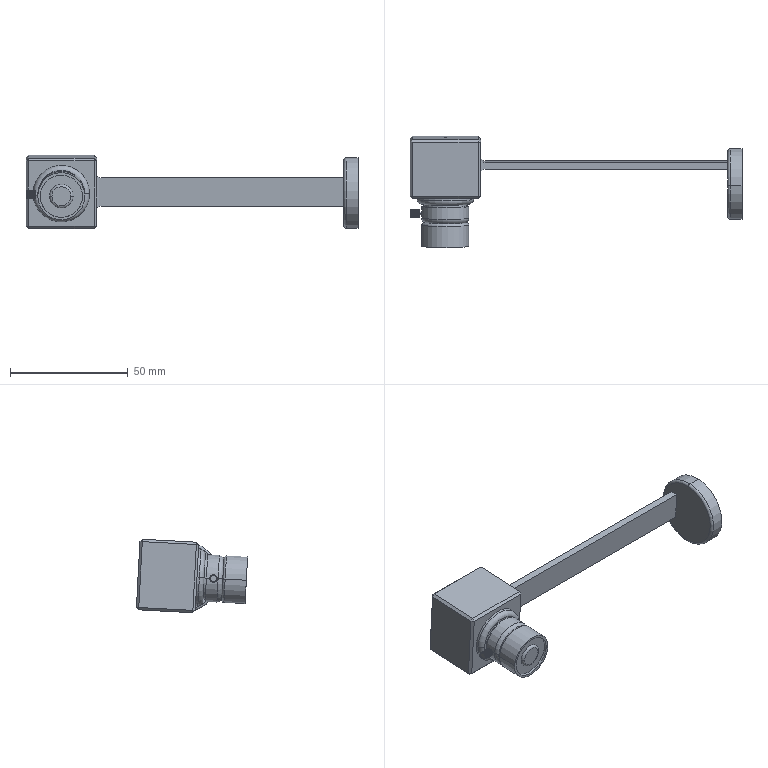Component | SolidWorks | Camera-1 | 1 solid | 164 faces | volume 37003 mm3 | plane 107 | cylinder 47 | torus 10 | commonest cylinder face diameters 2.8 x31 18 x4 20 x4 3 x2 24 x2 30 x2 1 x2